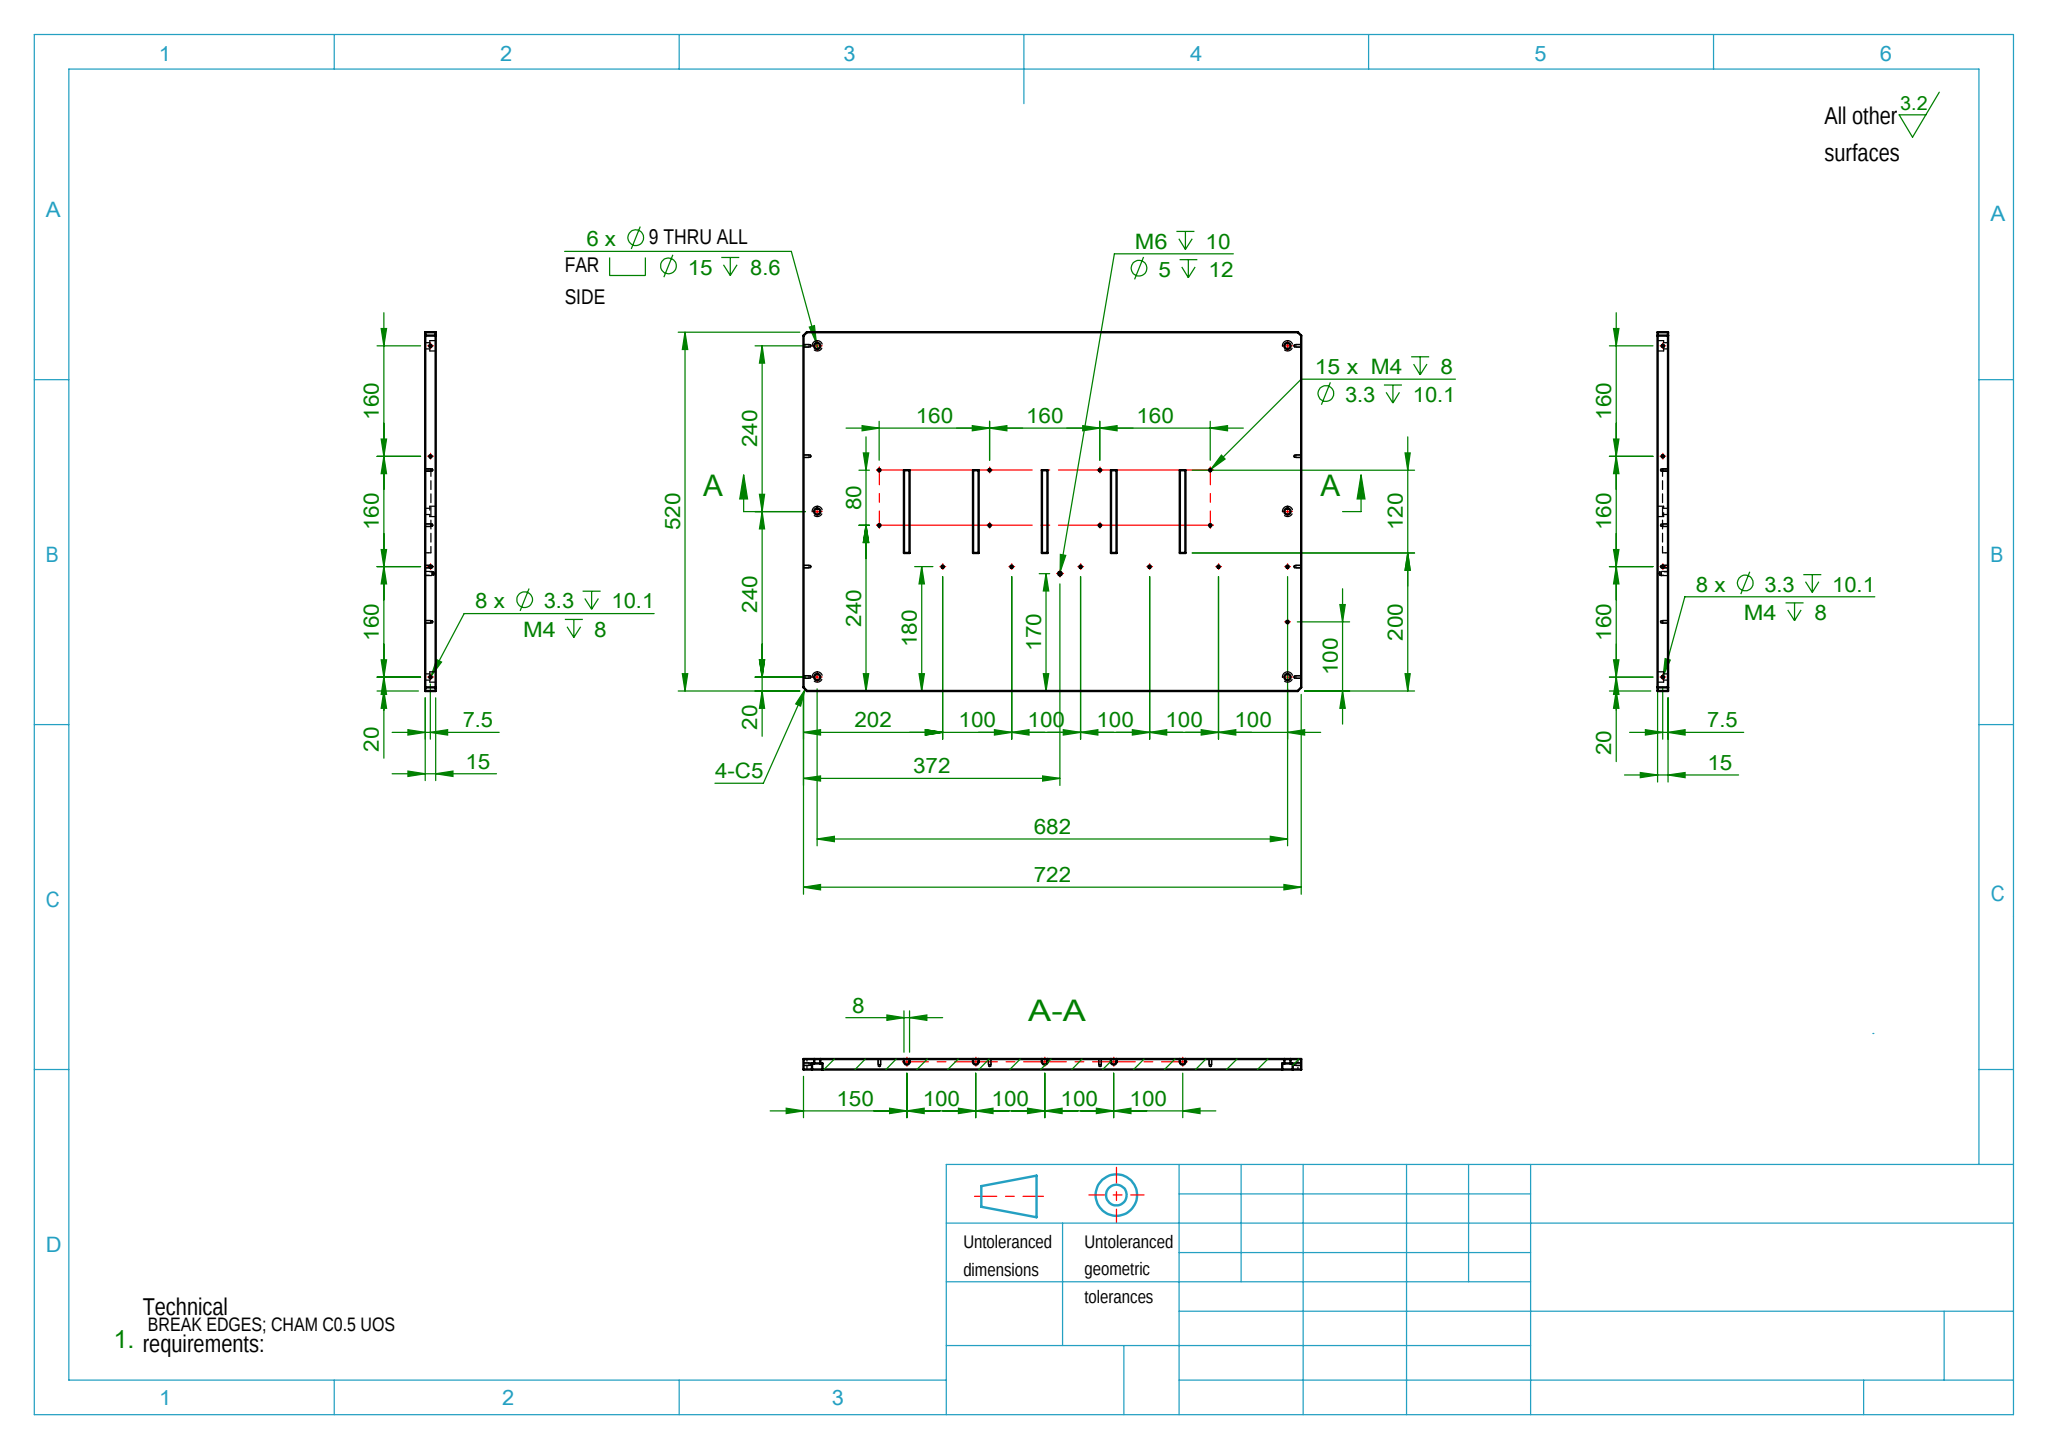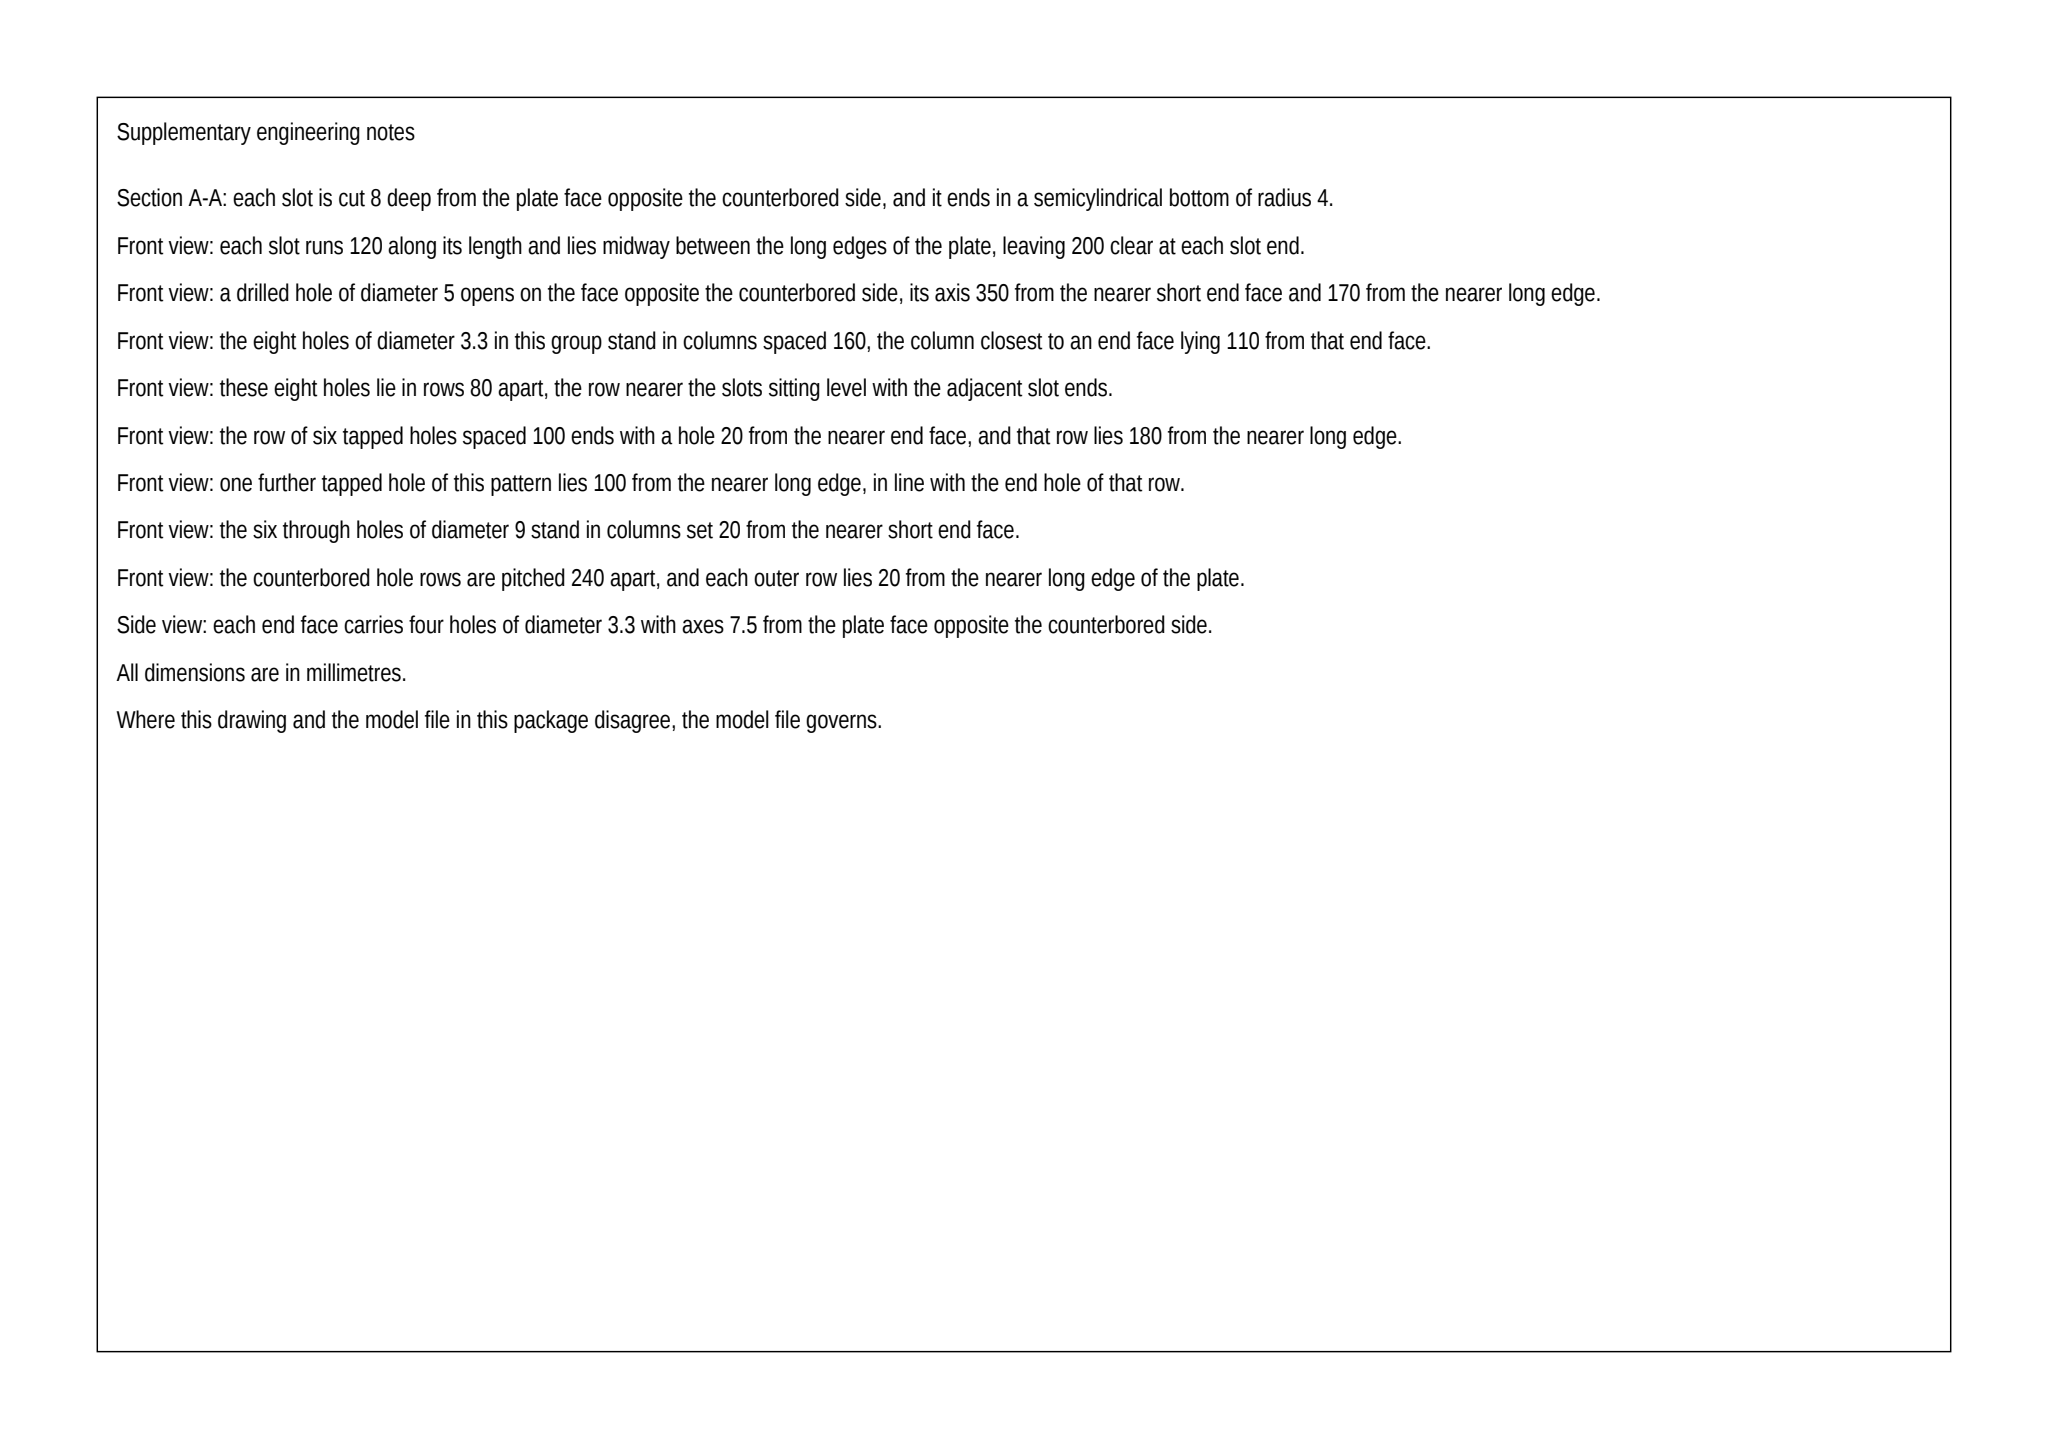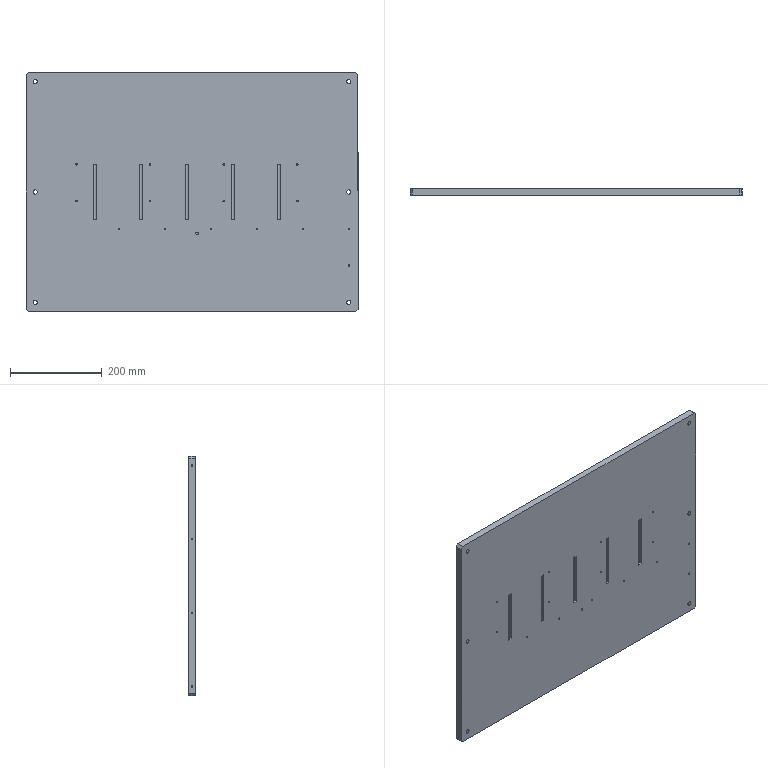Part | SolidWorks | mm | 1 solid | 161 faces | box 722 x 15 x 520 mm | volume 5582712 mm3 | cylinder 77 | cone 48 | plane 36 | commonest cylinder face diameters 3.3 x46 15 x12 9 x12 8 x5 5 x2
Drawing notes:
5X SLOT 8 WIDE X 120 LONG, R4 ENDS, DEPTH 8 FROM FRONT FACE (Y=0); SLOT CENTERLINES AT X=150, 250, 350, 450, 550 FROM LEFT EDGE, SLOTS SPAN Z=200 TO Z=320 FROM BOTTOM EDGE | from the solid: cylinders dia 8, axis z, pos [150/250/350/450/550, y=4.0], length 120; axis_planes z=200 (5) and z=320 (5); y planes 0 and 15 (plate thickness 15)
6X M4 DP 8, DRILL Ø3.3 DP 10.1 IN FRONT FACE, ROW AT Z=180 FROM BOTTOM EDGE; X=202, 302, 402, 502, 602, 702 FROM LEFT EDGE | from the solid: cylinders dia 3.3, axis y, pos [202/302/402/502/602/702, z=180], length 10.1
8X M4 DP 8, DRILL Ø3.3 DP 10.1 IN FRONT FACE, TWO ROWS AT Z=240 AND Z=320 FROM BOTTOM EDGE; X=110, 270, 430, 590 FROM LEFT EDGE | from the solid: cylinders dia 3.3, axis y, pos [110/270/430/590, z=240] and [110/270/430/590, z=320], length 10.1
ALL DIMENSIONS IN MILLIMETERS | from the solid: STEP model facts stated in mm (bbox_xyz 722 x 15 x 520 mm)
6X Ø9 THRU FROM FRONT FACE, C'BORE Ø15 DP 8.6 FROM BACK FACE; AT X=20 AND X=702, Z=20, 260 AND 500 FROM BOTTOM-LEFT CORNER | from the solid: cylinders dia 9.0 axis y len 6.4 and dia 15.0 axis y len 8.6 at (20/702, Z=20/260/500)
5X SLOT 8 WIDE, R4 ROUND ENDS, SLOT AXIS AT Y=4 FROM FRONT FACE (DEPTH 8); SLOT ENDS AT Z=200 AND Z=320 FROM BOTTOM EDGE | from the solid: cylinders dia 8.0 axis z, y=4.0, len 120 at X=150/250/350/450/550; planes z=200 and z=320
8X M4 DP 8, DRILL Ø3.3 DP 10.1 IN BOTH SIDE FACES (X=0 AND X=722), AT Y=7.5 FROM FRONT FACE; Z=20, 180, 340, 500 FROM BOTTOM EDGE | from the solid: cylinders dia 3.3 axis x, y=7.5, Z=20/180/340/500, len 10.1
build123d program:
from build123d import *

# Parameters (mm, degrees)
SKETCH1_W                                       = 722
SKETCH1_H                                       = 520
BOSS_EXTRUDE1_DEPTH                             = 15
M8_HEX_SOCKET_HEAD_CAP_SCREW_CBORE1_D           = 9
M8_HEX_SOCKET_HEAD_CAP_SCREW_CBORE1_CBORE_D     = 15
M8_HEX_SOCKET_HEAD_CAP_SCREW_CBORE1_CBORE_DEPTH = 8.6
CUT_EXTRUDE1_DEPTH                              = 60
LPATTERN1_COUNT                                 = 3
LPATTERN1_PITCH                                 = 100
LPATTERN2_COUNT                                 = 3
LPATTERN2_PITCH                                 = 100
M4_TAPPED_HOLE1_D                               = 3.3
M4_TAPPED_HOLE1_DEPTH                           = 10.1
M4_TAPPED_HOLE1_TIP                             = 0.9914
M6_TAPPED_HOLE1_D                               = 5
M6_TAPPED_HOLE1_DEPTH                           = 12
M6_TAPPED_HOLE1_TIP                             = 1.502
CHAMFER1_SIZE                                   = 5
M4_TAPPED_HOLE3_AT_2_COUNT                      = 2
M4_TAPPED_HOLE3_AT_2_PITCH                      = 160
M4_TAPPED_HOLE3_AT_3_COUNT                      = 2
M4_TAPPED_HOLE3_AT_3_PITCH                      = 320
M4_TAPPED_HOLE3_AT_4_COUNT                      = 2
M4_TAPPED_HOLE3_AT_4_PITCH                      = 480


with BuildPart() as part:
    # Sketch1 → Boss-Extrude1 (new body)
    with BuildSketch(Plane(origin=(0, 0, 0), x_dir=(1, 0, 0), z_dir=(0, 1, 0))):
        with Locations((361, 260)):
            Rectangle(SKETCH1_W, SKETCH1_H)
    extrude(amount=BOSS_EXTRUDE1_DEPTH)

    # M8 Hex Socket Head Cap Screw CBORE1 (through all)
    with Locations(Plane(origin=(0, 15, 0), x_dir=(1, 0, 0), z_dir=(0, 1, 0))):
        with Locations((702, 20), (702, 260), (702, 500), (20, 500), (20, 260), (20, 20)):
            CounterBoreHole(M8_HEX_SOCKET_HEAD_CAP_SCREW_CBORE1_D / 2, M8_HEX_SOCKET_HEAD_CAP_SCREW_CBORE1_CBORE_D / 2, M8_HEX_SOCKET_HEAD_CAP_SCREW_CBORE1_CBORE_DEPTH)

    # Sketch4 → Cut-Extrude1 (cut, symmetric)
    with BuildSketch(Plane.XY.offset(-260)):
        with BuildLine():
            Line((354, 0), (346, 0))
            Line((346, 0), (346, 4))
            ThreePointArc((346, 4), (350, 8), (354, 4))
            Line((354, 4), (354, 0))
        make_face()
    cut_extrude1 = extrude(amount=CUT_EXTRUDE1_DEPTH, both=True, mode=Mode.SUBTRACT)

    # LPattern1: Cut-Extrude1 ×3
    with Locations(*[(-i * LPATTERN1_PITCH, 0, 0) for i in range(1, LPATTERN1_COUNT)]):
        add(cut_extrude1, mode=Mode.SUBTRACT)

    # LPattern2: Cut-Extrude1 ×3
    with Locations(*[(i * LPATTERN2_PITCH, 0, 0) for i in range(1, LPATTERN2_COUNT)]):
        add(cut_extrude1, mode=Mode.SUBTRACT)

    # M4 Tapped Hole1
    with Locations(Plane(origin=(0, 0, 0), x_dir=(-1, 0, 0), z_dir=(0, -1, 0))):
        with Locations((-590, 200), (-590, 280), (-430, 280), (-430, 200), (-270, 200), (-270, 280), (-110, 280), (-110, 200), (-502, 340), (-402, 340), (-302, 340), (-202, 340), (-602, 340), (-702, 340), (-702, 420)):
            Hole(M4_TAPPED_HOLE1_D / 2, depth=M4_TAPPED_HOLE1_DEPTH)
            with Locations((0, 0, -(M4_TAPPED_HOLE1_DEPTH + M4_TAPPED_HOLE1_TIP / 2))):  # 118° drill point
                Cone(0, M4_TAPPED_HOLE1_D / 2, M4_TAPPED_HOLE1_TIP, mode=Mode.SUBTRACT)

    # M6 Tapped Hole1
    with Locations(Plane(origin=(0, 0, 0), x_dir=(-1, 0, 0), z_dir=(0, -1, 0))):
        with Locations((-372, 350)):
            Hole(M6_TAPPED_HOLE1_D / 2, depth=M6_TAPPED_HOLE1_DEPTH)
            with Locations((0, 0, -(M6_TAPPED_HOLE1_DEPTH + M6_TAPPED_HOLE1_TIP / 2))):  # 118° drill point
                Cone(0, M6_TAPPED_HOLE1_D / 2, M6_TAPPED_HOLE1_TIP, mode=Mode.SUBTRACT)

    # Chamfer1
    chamfer1_edges = [part.edges().sort_by_distance(p)[0] for p in [
        (0, 7.5, -520),
        (722, 7.5, -520),
        (722, 7.5, 0),
        (0, 7.5, 0),
    ]]
    chamfer(chamfer1_edges, length=CHAMFER1_SIZE)

    # Sketch12 → M4 Tapped Hole3 (revolve, cut)
    with BuildSketch(Plane(origin=(0, 7.5, -500), x_dir=(0, 0, 1), z_dir=(0, 1, 0))):
        Polygon((0, 0), (0, 11.091), (1.65, 10.1), (1.65, 0), align=None)
    m4_tapped_hole3 = revolve(axis=Axis((-6.35, 7.5, -500), (1, 0, 0)), mode=Mode.SUBTRACT)

    # M4 Tapped Hole3 at 2: M4 Tapped Hole3 ×2
    with Locations(*[(0, 0, i * M4_TAPPED_HOLE3_AT_2_PITCH) for i in range(1, M4_TAPPED_HOLE3_AT_2_COUNT)]):
        add(m4_tapped_hole3, mode=Mode.SUBTRACT)

    # M4 Tapped Hole3 at 3: M4 Tapped Hole3 ×2
    with Locations(*[(0, 0, i * M4_TAPPED_HOLE3_AT_3_PITCH) for i in range(1, M4_TAPPED_HOLE3_AT_3_COUNT)]):
        add(m4_tapped_hole3, mode=Mode.SUBTRACT)

    # M4 Tapped Hole3 at 4: M4 Tapped Hole3 ×2
    with Locations(*[(0, 0, i * M4_TAPPED_HOLE3_AT_4_PITCH) for i in range(1, M4_TAPPED_HOLE3_AT_4_COUNT)]):
        add(m4_tapped_hole3, mode=Mode.SUBTRACT)

    # Mirror1: M4 Tapped Hole3 across plane
    add(m4_tapped_hole3.mirror(Plane(origin=(361, 0, 0), x_dir=(0, 0, 1), z_dir=(1, 0, 0))), mode=Mode.SUBTRACT)

    # Mirror1 copy 1 sketch → Mirror1 copy 1 (revolve, cut)
    with BuildSketch(Plane(origin=(722, 7.5, -340), x_dir=(0, 0, 1), z_dir=(0, 1, 0))):
        Polygon((0, 0), (0, -11.091), (1.65, -10.1), (1.65, 0), align=None)
    revolve(axis=Axis((728.35, 7.5, -340), (1, 0, 0)), mode=Mode.SUBTRACT)

    # Mirror1 copy 2 sketch → Mirror1 copy 2 (revolve, cut)
    with BuildSketch(Plane(origin=(722, 7.5, -180), x_dir=(0, 0, 1), z_dir=(0, 1, 0))):
        Polygon((0, 0), (0, -11.091), (1.65, -10.1), (1.65, 0), align=None)
    revolve(axis=Axis((728.35, 7.5, -180), (1, 0, 0)), mode=Mode.SUBTRACT)

    # Mirror1 copy 3 sketch → Mirror1 copy 3 (revolve, cut)
    with BuildSketch(Plane(origin=(722, 7.5, -20), x_dir=(0, 0, 1), z_dir=(0, 1, 0))):
        Polygon((0, 0), (0, -11.091), (1.65, -10.1), (1.65, 0), align=None)
    revolve(axis=Axis((728.35, 7.5, -20), (1, 0, 0)), mode=Mode.SUBTRACT)


solid = part.part